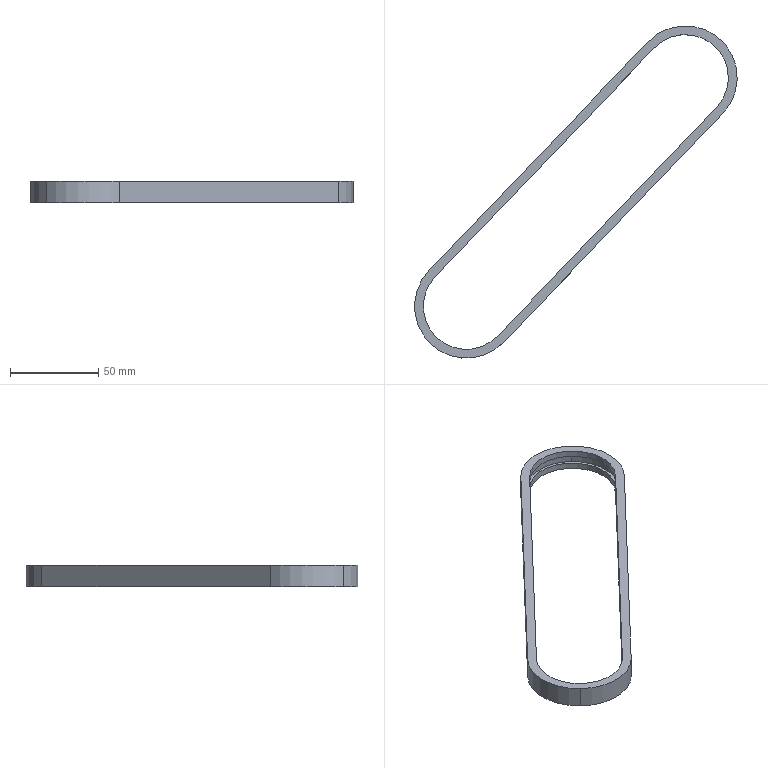Component | SolidWorks | LD101-02-Chain35B-2-1 | 1 solid | 24 faces | box 183.32 x 188.82 x 12 mm | volume 27813 mm3 | cylinder 12 | plane 12 | commonest cylinder face diameters 48.82 x6 52 x3 58.82 x3 | material 45
build123d program:
from build123d import *

# Parameters (mm, degrees)
EXTRUDE_THIN1_DEPTH            = 6
CHAIN_PLATE_GAP_SPROCKET_DEPTH = 2.385


with BuildPart() as part:
    # Sketch1_2 → Extrude-Thin1 (new, symmetric)
    with BuildSketch(Plane.XY):
        with BuildLine():
            Line((90, 29.41), (-90, 29.41))
            ThreePointArc((-90, 29.41), (-119.41, 0), (-90, -29.41))
            Line((-90, -29.41), (90, -29.41))
            ThreePointArc((90, -29.41), (119.41, 0), (90, 29.41))
        make_face()
        with BuildLine():
            Line((90, 24.41), (-90, 24.41))
            ThreePointArc((-90, 24.41), (-114.41, 0), (-90, -24.41))
            Line((-90, -24.41), (90, -24.41))
            ThreePointArc((90, -24.41), (114.41, 0), (90, 24.41))
        make_face(mode=Mode.SUBTRACT)
    extrude(amount=EXTRUDE_THIN1_DEPTH, both=True)

    # Sketch1_2 2 → Chain Plate Gap-Sprocket (cut, symmetric)
    with BuildSketch(Plane.XY):
        with BuildLine():
            Line((90, 26), (-90, 26))
            ThreePointArc((-90, 26), (-116, 0), (-90, -26))
            Line((-90, -26), (90, -26))
            ThreePointArc((90, -26), (116, 0), (90, 26))
        make_face()
        with BuildLine():
            Line((90, 22.82), (-90, 22.82))
            ThreePointArc((-90, 22.82), (-112.82, 0), (-90, -22.82))
            Line((-90, -22.82), (90, -22.82))
            ThreePointArc((90, -22.82), (112.82, 0), (90, 22.82))
        make_face(mode=Mode.SUBTRACT)
    extrude(amount=CHAIN_PLATE_GAP_SPROCKET_DEPTH, both=True, mode=Mode.SUBTRACT)


solid = part.part

# Placed as in the assembly
solid = solid.moved(Location((309.461, -246.897, 314.107), (0, 0, -133.762)))
STEP:
#1=COLOUR_RGB('',0.7922,0.8196,0.9333);
#2=FILL_AREA_STYLE_COLOUR('',#1);
#3=FILL_AREA_STYLE('',(#2));
#4=SURFACE_STYLE_FILL_AREA(#3);
#5=SURFACE_SIDE_STYLE('',(#4));
#6=SURFACE_STYLE_USAGE(.BOTH.,#5);
#7=PRESENTATION_STYLE_ASSIGNMENT((#6));
#8=CARTESIAN_POINT('',(15.342,-6.422,12.273));
#9=VERTEX_POINT('',#8);
#10=CARTESIAN_POINT('',(13.895,-6.453,12.273));
#11=VERTEX_POINT('',#10);
#12=CARTESIAN_POINT('',(14.634,-7.161,12.273));
#13=DIRECTION('',(0.,0.,1.));
#14=DIRECTION('',(-0.6917,-0.7222,0.));
#15=AXIS2_PLACEMENT_3D('',#12,#13,#14);
#16=CIRCLE('',#15,1.024);
#17=EDGE_CURVE('',#9,#11,#16,.T.);
#18=ORIENTED_EDGE('',*,*,#17,.F.);
#19=CARTESIAN_POINT('',(15.342,-6.422,12.46));
#20=VERTEX_POINT('',#19);
#21=CARTESIAN_POINT('',(15.342,-6.422,12.273));
#22=DIRECTION('',(0.,0.,1.));
#23=VECTOR('',#22,39.37);
#24=LINE('',#21,#23);
#25=EDGE_CURVE('',#9,#20,#24,.T.);
#26=ORIENTED_EDGE('',*,*,#25,.T.);
#27=CARTESIAN_POINT('',(13.895,-6.453,12.46));
#28=VERTEX_POINT('',#27);
#29=CARTESIAN_POINT('',(14.634,-7.161,12.46));
#30=DIRECTION('',(0.,0.,1.));
#31=DIRECTION('',(-0.6917,-0.7222,0.));
#32=AXIS2_PLACEMENT_3D('',#29,#30,#31);
#33=CIRCLE('',#32,1.024);
#34=EDGE_CURVE('',#20,#28,#33,.T.);
#35=ORIENTED_EDGE('',*,*,#34,.T.);
#36=CARTESIAN_POINT('',(13.895,-6.453,12.273));
#37=DIRECTION('',(0.,0.,1.));
#38=VECTOR('',#37,39.37);
#39=LINE('',#36,#38);
#40=EDGE_CURVE('',#11,#28,#39,.T.);
#41=ORIENTED_EDGE('',*,*,#40,.F.);
#42=EDGE_LOOP('',(#18,#26,#35,#41));
#43=FACE_OUTER_BOUND('',#42,.T.);
#44=CARTESIAN_POINT('',(14.634,-7.161,12.273));
#45=DIRECTION('',(0.,0.,1.));
#46=DIRECTION('',(0.6917,0.7222,0.));
#47=AXIS2_PLACEMENT_3D('',#44,#45,#46);
#48=CYLINDRICAL_SURFACE('',#47,1.024);
#49=ADVANCED_FACE('',(#43),#48,.F.);
#50=CARTESIAN_POINT('',(9.068,-12.973,12.273));
#51=VERTEX_POINT('',#50);
#52=CARTESIAN_POINT('',(9.039,-11.615,12.273));
#53=VERTEX_POINT('',#52);
#54=CARTESIAN_POINT('',(9.733,-12.279,12.273));
#55=DIRECTION('',(0.,0.,-1.));
#56=DIRECTION('',(-0.6917,-0.7222,0.));
#57=AXIS2_PLACEMENT_3D('',#54,#55,#56);
#58=CIRCLE('',#57,0.961);
#59=EDGE_CURVE('',#51,#53,#58,.T.);
#60=ORIENTED_EDGE('',*,*,#59,.F.);
#61=CARTESIAN_POINT('',(9.068,-12.973,12.13));
#62=VERTEX_POINT('',#61);
#63=CARTESIAN_POINT('',(9.068,-12.973,12.603));
#64=DIRECTION('',(0.,0.,-1.));
#65=VECTOR('',#64,39.37);
#66=LINE('',#63,#65);
#67=EDGE_CURVE('',#51,#62,#66,.T.);
#68=ORIENTED_EDGE('',*,*,#67,.T.);
#69=CARTESIAN_POINT('',(9.039,-11.615,12.13));
#70=VERTEX_POINT('',#69);
#71=CARTESIAN_POINT('',(9.733,-12.279,12.13));
#72=DIRECTION('',(0.,0.,1.));
#73=DIRECTION('',(0.6917,0.7222,0.));
#74=AXIS2_PLACEMENT_3D('',#71,#72,#73);
#75=CIRCLE('',#74,0.961);
#76=EDGE_CURVE('',#70,#62,#75,.T.);
#77=ORIENTED_EDGE('',*,*,#76,.F.);
#78=CARTESIAN_POINT('',(9.039,-11.615,12.603));
#79=DIRECTION('',(0.,0.,-1.));
#80=VECTOR('',#79,39.37);
#81=LINE('',#78,#80);
#82=EDGE_CURVE('',#53,#70,#81,.T.);
#83=ORIENTED_EDGE('',*,*,#82,.F.);
#84=EDGE_LOOP('',(#60,#68,#77,#83));
#85=FACE_OUTER_BOUND('',#84,.T.);
#86=CARTESIAN_POINT('',(9.733,-12.279,12.603));
#87=DIRECTION('',(0.,0.,-1.));
#88=DIRECTION('',(-0.6917,-0.7222,0.));
#89=AXIS2_PLACEMENT_3D('',#86,#87,#88);
#90=CYLINDRICAL_SURFACE('',#89,0.961);
#91=ADVANCED_FACE('',(#85),#90,.F.);
#92=CARTESIAN_POINT('',(8.932,-13.116,12.603));
#93=VERTEX_POINT('',#92);
#94=CARTESIAN_POINT('',(10.569,-13.08,12.603));
#95=VERTEX_POINT('',#94);
#96=CARTESIAN_POINT('',(9.733,-12.279,12.603));
#97=DIRECTION('',(0.,0.,1.));
#98=DIRECTION('',(-0.6917,-0.7222,0.));
#99=AXIS2_PLACEMENT_3D('',#96,#97,#98);
#100=CIRCLE('',#99,1.158);
#101=EDGE_CURVE('',#93,#95,#100,.T.);
#102=ORIENTED_EDGE('',*,*,#101,.F.);
#103=CARTESIAN_POINT('',(8.932,-13.116,12.13));
#104=VERTEX_POINT('',#103);
#105=CARTESIAN_POINT('',(8.932,-13.116,12.603));
#106=DIRECTION('',(0.,0.,-1.));
#107=VECTOR('',#106,39.37);
#108=LINE('',#105,#107);
#109=EDGE_CURVE('',#93,#104,#108,.T.);
#110=ORIENTED_EDGE('',*,*,#109,.T.);
#111=CARTESIAN_POINT('',(10.569,-13.08,12.13));
#112=VERTEX_POINT('',#111);
#113=CARTESIAN_POINT('',(9.733,-12.279,12.13));
#114=DIRECTION('',(0.,0.,1.));
#115=DIRECTION('',(-0.6917,-0.7222,0.));
#116=AXIS2_PLACEMENT_3D('',#113,#114,#115);
#117=CIRCLE('',#116,1.158);
#118=EDGE_CURVE('',#104,#112,#117,.T.);
#119=ORIENTED_EDGE('',*,*,#118,.T.);
#120=CARTESIAN_POINT('',(10.569,-13.08,12.603));
#121=DIRECTION('',(0.,0.,-1.));
#122=VECTOR('',#121,39.37);
#123=LINE('',#120,#122);
#124=EDGE_CURVE('',#95,#112,#123,.T.);
#125=ORIENTED_EDGE('',*,*,#124,.F.);
#126=EDGE_LOOP('',(#102,#110,#119,#125));
#127=FACE_OUTER_BOUND('',#126,.T.);
#128=CARTESIAN_POINT('',(9.733,-12.279,12.603));
#129=DIRECTION('',(0.,0.,-1.));
#130=DIRECTION('',(-0.6917,-0.7222,0.));
#131=AXIS2_PLACEMENT_3D('',#128,#129,#130);
#132=CYLINDRICAL_SURFACE('',#131,1.158);
#133=ADVANCED_FACE('',(#127),#132,.T.);
#134=CARTESIAN_POINT('',(9.039,-11.615,12.603));
#135=VERTEX_POINT('',#134);
#136=CARTESIAN_POINT('',(9.068,-12.973,12.603));
#137=VERTEX_POINT('',#136);
#138=CARTESIAN_POINT('',(9.733,-12.279,12.603));
#139=DIRECTION('',(0.,0.,1.));
#140=DIRECTION('',(0.6917,0.7222,0.));
#141=AXIS2_PLACEMENT_3D('',#138,#139,#140);
#142=CIRCLE('',#141,0.961);
#143=EDGE_CURVE('',#135,#137,#142,.T.);
#144=ORIENTED_EDGE('',*,*,#143,.T.);
#145=CARTESIAN_POINT('',(9.068,-12.973,12.46));
#146=VERTEX_POINT('',#145);
#147=CARTESIAN_POINT('',(9.068,-12.973,12.603));
#148=DIRECTION('',(0.,0.,-1.));
#149=VECTOR('',#148,39.37);
#150=LINE('',#147,#149);
#151=EDGE_CURVE('',#137,#146,#150,.T.);
#152=ORIENTED_EDGE('',*,*,#151,.T.);
#153=CARTESIAN_POINT('',(9.039,-11.615,12.46));
#154=VERTEX_POINT('',#153);
#155=CARTESIAN_POINT('',(9.733,-12.279,12.46));
#156=DIRECTION('',(0.,0.,-1.));
#157=DIRECTION('',(-0.6917,-0.7222,0.));
#158=AXIS2_PLACEMENT_3D('',#155,#156,#157);
#159=CIRCLE('',#158,0.961);
#160=EDGE_CURVE('',#146,#154,#159,.T.);
#161=ORIENTED_EDGE('',*,*,#160,.T.);
#162=CARTESIAN_POINT('',(9.039,-11.615,12.603));
#163=DIRECTION('',(0.,0.,-1.));
#164=VECTOR('',#163,39.37);
#165=LINE('',#162,#164);
#166=EDGE_CURVE('',#135,#154,#165,.T.);
#167=ORIENTED_EDGE('',*,*,#166,.F.);
#168=EDGE_LOOP('',(#144,#152,#161,#167));
#169=FACE_OUTER_BOUND('',#168,.T.);
#170=CARTESIAN_POINT('',(9.733,-12.279,12.603));
#171=DIRECTION('',(0.,0.,-1.));
#172=DIRECTION('',(-0.6917,-0.7222,0.));
#173=AXIS2_PLACEMENT_3D('',#170,#171,#172);
#174=CYLINDRICAL_SURFACE('',#173,0.961);
#175=ADVANCED_FACE('',(#169),#174,.F.);
#176=CARTESIAN_POINT('',(13.94,-6.497,12.603));
#177=VERTEX_POINT('',#176);
#178=CARTESIAN_POINT('',(13.94,-6.497,12.46));
#179=VERTEX_POINT('',#178);
#180=CARTESIAN_POINT('',(13.94,-6.497,12.603));
#181=DIRECTION('',(0.,0.,-1.));
#182=VECTOR('',#181,39.37);
#183=LINE('',#180,#182);
#184=EDGE_CURVE('',#177,#179,#183,.T.);
#185=ORIENTED_EDGE('',*,*,#184,.T.);
#186=CARTESIAN_POINT('',(15.328,-7.826,12.46));
#187=VERTEX_POINT('',#186);
#188=CARTESIAN_POINT('',(14.634,-7.161,12.46));
#189=DIRECTION('',(0.,0.,-1.));
#190=DIRECTION('',(-0.6917,-0.7222,0.));
#191=AXIS2_PLACEMENT_3D('',#188,#189,#190);
#192=CIRCLE('',#191,0.961);
#193=EDGE_CURVE('',#179,#187,#192,.T.);
#194=ORIENTED_EDGE('',*,*,#193,.T.);
#195=CARTESIAN_POINT('',(15.328,-7.826,12.603));
#196=VERTEX_POINT('',#195);
#197=CARTESIAN_POINT('',(15.328,-7.826,12.603));
#198=DIRECTION('',(0.,0.,-1.));
#199=VECTOR('',#198,39.37);
#200=LINE('',#197,#199);
#201=EDGE_CURVE('',#196,#187,#200,.T.);
#202=ORIENTED_EDGE('',*,*,#201,.F.);
#203=CARTESIAN_POINT('',(14.634,-7.161,12.603));
#204=DIRECTION('',(0.,0.,1.));
#205=DIRECTION('',(-0.6917,-0.7222,0.));
#206=AXIS2_PLACEMENT_3D('',#203,#204,#205);
#207=CIRCLE('',#206,0.961);
#208=EDGE_CURVE('',#196,#177,#207,.T.);
#209=ORIENTED_EDGE('',*,*,#208,.T.);
#210=EDGE_LOOP('',(#185,#194,#202,#209));
#211=FACE_OUTER_BOUND('',#210,.T.);
#212=CARTESIAN_POINT('',(14.634,-7.161,12.603));
#213=DIRECTION('',(0.,0.,-1.));
#214=DIRECTION('',(-0.6917,-0.7222,0.));
#215=AXIS2_PLACEMENT_3D('',#212,#213,#214);
#216=CYLINDRICAL_SURFACE('',#215,0.961);
#217=ADVANCED_FACE('',(#211),#216,.F.);
#218=ORIENTED_EDGE('',*,*,#166,.T.);
#219=CARTESIAN_POINT('',(13.94,-6.497,12.46));
#220=DIRECTION('',(0.6917,0.7222,0.));
#221=VECTOR('',#220,39.37);
#222=LINE('',#219,#221);
#223=EDGE_CURVE('',#154,#179,#222,.T.);
#224=ORIENTED_EDGE('',*,*,#223,.T.);
#225=ORIENTED_EDGE('',*,*,#184,.F.);
#226=CARTESIAN_POINT('',(13.94,-6.497,12.603));
#227=DIRECTION('',(-0.6917,-0.7222,0.));
#228=VECTOR('',#227,39.37);
#229=LINE('',#226,#228);
#230=EDGE_CURVE('',#177,#135,#229,.T.);
#231=ORIENTED_EDGE('',*,*,#230,.T.);
#232=EDGE_LOOP('',(#218,#224,#225,#231));
#233=FACE_OUTER_BOUND('',#232,.T.);
#234=CARTESIAN_POINT('',(13.94,-6.497,12.603));
#235=DIRECTION('',(0.7222,-0.6917,0.));
#236=DIRECTION('',(0.,0.,-1.));
#237=AXIS2_PLACEMENT_3D('',#234,#235,#236);
#238=PLANE('',#237);
#239=ADVANCED_FACE('',(#233),#238,.T.);
#240=ORIENTED_EDGE('',*,*,#151,.F.);
#241=CARTESIAN_POINT('',(10.427,-12.944,12.603));
#242=VERTEX_POINT('',#241);
#243=CARTESIAN_POINT('',(9.733,-12.279,12.603));
#244=DIRECTION('',(0.,0.,1.));
#245=DIRECTION('',(0.6917,0.7222,0.));
#246=AXIS2_PLACEMENT_3D('',#243,#244,#245);
#247=CIRCLE('',#246,0.961);
#248=EDGE_CURVE('',#137,#242,#247,.T.);
#249=ORIENTED_EDGE('',*,*,#248,.T.);
#250=CARTESIAN_POINT('',(10.427,-12.944,12.46));
#251=VERTEX_POINT('',#250);
#252=CARTESIAN_POINT('',(10.427,-12.944,12.603));
#253=DIRECTION('',(0.,0.,-1.));
#254=VECTOR('',#253,39.37);
#255=LINE('',#252,#254);
#256=EDGE_CURVE('',#242,#251,#255,.T.);
#257=ORIENTED_EDGE('',*,*,#256,.T.);
#258=CARTESIAN_POINT('',(9.733,-12.279,12.46));
#259=DIRECTION('',(0.,0.,-1.));
#260=DIRECTION('',(-0.6917,-0.7222,0.));
#261=AXIS2_PLACEMENT_3D('',#258,#259,#260);
#262=CIRCLE('',#261,0.961);
#263=EDGE_CURVE('',#251,#146,#262,.T.);
#264=ORIENTED_EDGE('',*,*,#263,.T.);
#265=EDGE_LOOP('',(#240,#249,#257,#264));
#266=FACE_OUTER_BOUND('',#265,.T.);
#267=CARTESIAN_POINT('',(9.733,-12.279,12.603));
#268=DIRECTION('',(0.,0.,-1.));
#269=DIRECTION('',(-0.6917,-0.7222,0.));
#270=AXIS2_PLACEMENT_3D('',#267,#268,#269);
#271=CYLINDRICAL_SURFACE('',#270,0.961);
#272=ADVANCED_FACE('',(#266),#271,.F.);
#273=ORIENTED_EDGE('',*,*,#201,.T.);
#274=CARTESIAN_POINT('',(10.427,-12.944,12.46));
#275=DIRECTION('',(-0.6917,-0.7222,0.));
#276=VECTOR('',#275,39.37);
#277=LINE('',#274,#276);
#278=EDGE_CURVE('',#187,#251,#277,.T.);
#279=ORIENTED_EDGE('',*,*,#278,.T.);
#280=ORIENTED_EDGE('',*,*,#256,.F.);
#281=CARTESIAN_POINT('',(10.427,-12.944,12.603));
#282=DIRECTION('',(0.6917,0.7222,0.));
#283=VECTOR('',#282,39.37);
#284=LINE('',#281,#283);
#285=EDGE_CURVE('',#242,#196,#284,.T.);
#286=ORIENTED_EDGE('',*,*,#285,.T.);
#287=EDGE_LOOP('',(#273,#279,#280,#286));
#288=FACE_OUTER_BOUND('',#287,.T.);
#289=CARTESIAN_POINT('',(10.427,-12.944,12.603));
#290=DIRECTION('',(-0.7222,0.6917,0.));
#291=DIRECTION('',(0.,0.,1.));
#292=AXIS2_PLACEMENT_3D('',#289,#290,#291);
#293=PLANE('',#292);
#294=ADVANCED_FACE('',(#288),#293,.T.);
#295=CARTESIAN_POINT('',(15.471,-7.962,12.603));
#296=VERTEX_POINT('',#295);
#297=CARTESIAN_POINT('',(13.798,-6.36,12.603));
#298=VERTEX_POINT('',#297);
#299=CARTESIAN_POINT('',(14.634,-7.161,12.603));
#300=DIRECTION('',(0.,0.,1.));
#301=DIRECTION('',(-0.6917,-0.7222,0.));
#302=AXIS2_PLACEMENT_3D('',#299,#300,#301);
#303=CIRCLE('',#302,1.158);
#304=EDGE_CURVE('',#296,#298,#303,.T.);
#305=ORIENTED_EDGE('',*,*,#304,.T.);
#306=CARTESIAN_POINT('',(8.896,-11.479,12.603));
#307=VERTEX_POINT('',#306);
#308=CARTESIAN_POINT('',(13.798,-6.36,12.603));
#309=DIRECTION('',(-0.6917,-0.7222,0.));
#310=VECTOR('',#309,39.37);
#311=LINE('',#308,#310);
#312=EDGE_CURVE('',#298,#307,#311,.T.);
#313=ORIENTED_EDGE('',*,*,#312,.T.);
#314=CARTESIAN_POINT('',(9.733,-12.279,12.603));
#315=DIRECTION('',(0.,0.,1.));
#316=DIRECTION('',(-0.6917,-0.7222,0.));
#317=AXIS2_PLACEMENT_3D('',#314,#315,#316);
#318=CIRCLE('',#317,1.158);
#319=EDGE_CURVE('',#307,#93,#318,.T.);
#320=ORIENTED_EDGE('',*,*,#319,.T.);
#321=ORIENTED_EDGE('',*,*,#101,.T.);
#322=CARTESIAN_POINT('',(15.471,-7.962,12.603));
#323=DIRECTION('',(0.6917,0.7222,0.));
#324=VECTOR('',#323,39.37);
#325=LINE('',#322,#324);
#326=EDGE_CURVE('',#95,#296,#325,.T.);
#327=ORIENTED_EDGE('',*,*,#326,.T.);
#328=EDGE_LOOP('',(#305,#313,#320,#321,#327));
#329=FACE_OUTER_BOUND('',#328,.T.);
#330=ORIENTED_EDGE('',*,*,#208,.F.);
#331=ORIENTED_EDGE('',*,*,#285,.F.);
#332=ORIENTED_EDGE('',*,*,#248,.F.);
#333=ORIENTED_EDGE('',*,*,#143,.F.);
#334=ORIENTED_EDGE('',*,*,#230,.F.);
#335=EDGE_LOOP('',(#330,#331,#332,#333,#334));
#336=FACE_BOUND('',#335,.T.);
#337=CARTESIAN_POINT('',(14.634,-7.161,12.603));
#338=DIRECTION('',(0.,0.,-1.));
#339=DIRECTION('',(-0.6917,-0.7222,0.));
#340=AXIS2_PLACEMENT_3D('',#337,#338,#339);
#341=PLANE('',#340);
#342=ADVANCED_FACE('',(#329,#336),#341,.F.);
#343=CARTESIAN_POINT('',(15.471,-7.962,12.13));
#344=VERTEX_POINT('',#343);
#345=CARTESIAN_POINT('',(13.798,-6.36,12.13));
#346=VERTEX_POINT('',#345);
#347=CARTESIAN_POINT('',(14.634,-7.161,12.13));
#348=DIRECTION('',(0.,0.,1.));
#349=DIRECTION('',(-0.6917,-0.7222,0.));
#350=AXIS2_PLACEMENT_3D('',#347,#348,#349);
#351=CIRCLE('',#350,1.158);
#352=EDGE_CURVE('',#344,#346,#351,.T.);
#353=ORIENTED_EDGE('',*,*,#352,.F.);
#354=CARTESIAN_POINT('',(15.471,-7.962,12.13));
#355=DIRECTION('',(0.6917,0.7222,0.));
#356=VECTOR('',#355,39.37);
#357=LINE('',#354,#356);
#358=EDGE_CURVE('',#112,#344,#357,.T.);
#359=ORIENTED_EDGE('',*,*,#358,.F.);
#360=ORIENTED_EDGE('',*,*,#118,.F.);
#361=CARTESIAN_POINT('',(8.896,-11.479,12.13));
#362=VERTEX_POINT('',#361);
#363=CARTESIAN_POINT('',(9.733,-12.279,12.13));
#364=DIRECTION('',(0.,0.,1.));
#365=DIRECTION('',(-0.6917,-0.7222,0.));
#366=AXIS2_PLACEMENT_3D('',#363,#364,#365);
#367=CIRCLE('',#366,1.158);
#368=EDGE_CURVE('',#362,#104,#367,.T.);
#369=ORIENTED_EDGE('',*,*,#368,.F.);
#370=CARTESIAN_POINT('',(13.798,-6.36,12.13));
#371=DIRECTION('',(-0.6917,-0.7222,0.));
#372=VECTOR('',#371,39.37);
#373=LINE('',#370,#372);
#374=EDGE_CURVE('',#346,#362,#373,.T.);
#375=ORIENTED_EDGE('',*,*,#374,.F.);
#376=EDGE_LOOP('',(#353,#359,#360,#369,#375));
#377=FACE_OUTER_BOUND('',#376,.T.);
#378=CARTESIAN_POINT('',(10.427,-12.944,12.13));
#379=VERTEX_POINT('',#378);
#380=CARTESIAN_POINT('',(15.328,-7.826,12.13));
#381=VERTEX_POINT('',#380);
#382=CARTESIAN_POINT('',(10.427,-12.944,12.13));
#383=DIRECTION('',(0.6917,0.7222,0.));
#384=VECTOR('',#383,39.37);
#385=LINE('',#382,#384);
#386=EDGE_CURVE('',#379,#381,#385,.T.);
#387=ORIENTED_EDGE('',*,*,#386,.T.);
#388=CARTESIAN_POINT('',(13.94,-6.497,12.13));
#389=VERTEX_POINT('',#388);
#390=CARTESIAN_POINT('',(14.634,-7.161,12.13));
#391=DIRECTION('',(0.,0.,1.));
#392=DIRECTION('',(-0.6917,-0.7222,0.));
#393=AXIS2_PLACEMENT_3D('',#390,#391,#392);
#394=CIRCLE('',#393,0.961);
#395=EDGE_CURVE('',#381,#389,#394,.T.);
#396=ORIENTED_EDGE('',*,*,#395,.T.);
#397=CARTESIAN_POINT('',(13.94,-6.497,12.13));
#398=DIRECTION('',(-0.6917,-0.7222,0.));
#399=VECTOR('',#398,39.37);
#400=LINE('',#397,#399);
#401=EDGE_CURVE('',#389,#70,#400,.T.);
#402=ORIENTED_EDGE('',*,*,#401,.T.);
#403=ORIENTED_EDGE('',*,*,#76,.T.);
#404=CARTESIAN_POINT('',(9.733,-12.279,12.13));
#405=DIRECTION('',(0.,0.,1.));
#406=DIRECTION('',(0.6917,0.7222,0.));
#407=AXIS2_PLACEMENT_3D('',#404,#405,#406);
#408=CIRCLE('',#407,0.961);
#409=EDGE_CURVE('',#62,#379,#408,.T.);
#410=ORIENTED_EDGE('',*,*,#409,.T.);
#411=EDGE_LOOP('',(#387,#396,#402,#403,#410));
#412=FACE_BOUND('',#411,.T.);
#413=CARTESIAN_POINT('',(14.634,-7.161,12.13));
#414=DIRECTION('',(0.,0.,-1.));
#415=DIRECTION('',(-0.6917,-0.7222,0.));
#416=AXIS2_PLACEMENT_3D('',#413,#414,#415);
#417=PLANE('',#416);
#418=ADVANCED_FACE('',(#377,#412),#417,.T.);
#419=ORIENTED_EDGE('',*,*,#352,.T.);
#420=CARTESIAN_POINT('',(13.798,-6.36,12.603));
#421=DIRECTION('',(0.,0.,-1.));
#422=VECTOR('',#421,39.37);
#423=LINE('',#420,#422);
#424=EDGE_CURVE('',#298,#346,#423,.T.);
#425=ORIENTED_EDGE('',*,*,#424,.F.);
#426=ORIENTED_EDGE('',*,*,#304,.F.);
#427=CARTESIAN_POINT('',(15.471,-7.962,12.603));
#428=DIRECTION('',(0.,0.,-1.));
#429=VECTOR('',#428,39.37);
#430=LINE('',#427,#429);
#431=EDGE_CURVE('',#296,#344,#430,.T.);
#432=ORIENTED_EDGE('',*,*,#431,.T.);
#433=EDGE_LOOP('',(#419,#425,#426,#432));
#434=FACE_OUTER_BOUND('',#433,.T.);
#435=CARTESIAN_POINT('',(14.634,-7.161,12.603));
#436=DIRECTION('',(0.,0.,-1.));
#437=DIRECTION('',(-0.6917,-0.7222,0.));
#438=AXIS2_PLACEMENT_3D('',#435,#436,#437);
#439=CYLINDRICAL_SURFACE('',#438,1.158);
#440=ADVANCED_FACE('',(#434),#439,.T.);
#441=ORIENTED_EDGE('',*,*,#374,.T.);
#442=CARTESIAN_POINT('',(8.896,-11.479,12.603));
#443=DIRECTION('',(0.,0.,-1.));
#444=VECTOR('',#443,39.37);
#445=LINE('',#442,#444);
#446=EDGE_CURVE('',#307,#362,#445,.T.);
#447=ORIENTED_EDGE('',*,*,#446,.F.);
#448=ORIENTED_EDGE('',*,*,#312,.F.);
#449=ORIENTED_EDGE('',*,*,#424,.T.);
#450=EDGE_LOOP('',(#441,#447,#448,#449));
#451=FACE_OUTER_BOUND('',#450,.T.);
#452=CARTESIAN_POINT('',(13.798,-6.36,12.603));
#453=DIRECTION('',(0.7222,-0.6917,0.));
#454=DIRECTION('',(0.,0.,-1.));
#455=AXIS2_PLACEMENT_3D('',#452,#453,#454);
#456=PLANE('',#455);
#457=ADVANCED_FACE('',(#451),#456,.F.);
#458=ORIENTED_EDGE('',*,*,#109,.F.);
#459=ORIENTED_EDGE('',*,*,#319,.F.);
#460=ORIENTED_EDGE('',*,*,#446,.T.);
#461=ORIENTED_EDGE('',*,*,#368,.T.);
#462=EDGE_LOOP('',(#458,#459,#460,#461));
#463=FACE_OUTER_BOUND('',#462,.T.);
#464=CARTESIAN_POINT('',(9.733,-12.279,12.603));
#465=DIRECTION('',(0.,0.,-1.));
#466=DIRECTION('',(-0.6917,-0.7222,0.));
#467=AXIS2_PLACEMENT_3D('',#464,#465,#466);
#468=CYLINDRICAL_SURFACE('',#467,1.158);
#469=ADVANCED_FACE('',(#463),#468,.T.);
#470=ORIENTED_EDGE('',*,*,#358,.T.);
#471=ORIENTED_EDGE('',*,*,#431,.F.);
#472=ORIENTED_EDGE('',*,*,#326,.F.);
#473=ORIENTED_EDGE('',*,*,#124,.T.);
#474=EDGE_LOOP('',(#470,#471,#472,#473));
#475=FACE_OUTER_BOUND('',#474,.T.);
#476=CARTESIAN_POINT('',(15.471,-7.962,12.603));
#477=DIRECTION('',(-0.7222,0.6917,0.));
#478=DIRECTION('',(0.,0.,1.));
#479=AXIS2_PLACEMENT_3D('',#476,#477,#478);
#480=PLANE('',#479);
#481=ADVANCED_FACE('',(#475),#480,.F.);
#482=CARTESIAN_POINT('',(13.94,-6.497,12.273));
#483=VERTEX_POINT('',#482);
#484=CARTESIAN_POINT('',(15.328,-7.826,12.273));
#485=VERTEX_POINT('',#484);
#486=CARTESIAN_POINT('',(14.634,-7.161,12.273));
#487=DIRECTION('',(0.,0.,-1.));
#488=DIRECTION('',(-0.6917,-0.7222,0.));
#489=AXIS2_PLACEMENT_3D('',#486,#487,#488);
#490=CIRCLE('',#489,0.961);
#491=EDGE_CURVE('',#483,#485,#490,.T.);
#492=ORIENTED_EDGE('',*,*,#491,.F.);
#493=CARTESIAN_POINT('',(13.94,-6.497,12.603));
#494=DIRECTION('',(0.,0.,-1.));
#495=VECTOR('',#494,39.37);
#496=LINE('',#493,#495);
#497=EDGE_CURVE('',#483,#389,#496,.T.);
#498=ORIENTED_EDGE('',*,*,#497,.T.);
#499=ORIENTED_EDGE('',*,*,#395,.F.);
#500=CARTESIAN_POINT('',(15.328,-7.826,12.603));
#501=DIRECTION('',(0.,0.,-1.));
#502=VECTOR('',#501,39.37);
#503=LINE('',#500,#502);
#504=EDGE_CURVE('',#485,#381,#503,.T.);
#505=ORIENTED_EDGE('',*,*,#504,.F.);
#506=EDGE_LOOP('',(#492,#498,#499,#505));
#507=FACE_OUTER_BOUND('',#506,.T.);
#508=CARTESIAN_POINT('',(14.634,-7.161,12.603));
#509=DIRECTION('',(0.,0.,-1.));
#510=DIRECTION('',(-0.6917,-0.7222,0.));
#511=AXIS2_PLACEMENT_3D('',#508,#509,#510);
#512=CYLINDRICAL_SURFACE('',#511,0.961);
#513=ADVANCED_FACE('',(#507),#512,.F.);
#514=CARTESIAN_POINT('',(13.94,-6.497,12.273));
#515=DIRECTION('',(0.6917,0.7222,0.));
#516=VECTOR('',#515,39.37);
#517=LINE('',#514,#516);
#518=EDGE_CURVE('',#53,#483,#517,.T.);
#519=ORIENTED_EDGE('',*,*,#518,.F.);
#520=ORIENTED_EDGE('',*,*,#82,.T.);
#521=ORIENTED_EDGE('',*,*,#401,.F.);
#522=ORIENTED_EDGE('',*,*,#497,.F.);
#523=EDGE_LOOP('',(#519,#520,#521,#522));
#524=FACE_OUTER_BOUND('',#523,.T.);
#525=CARTESIAN_POINT('',(13.94,-6.497,12.603));
#526=DIRECTION('',(0.7222,-0.6917,0.));
#527=DIRECTION('',(0.,0.,-1.));
#528=AXIS2_PLACEMENT_3D('',#525,#526,#527);
#529=PLANE('',#528);
#530=ADVANCED_FACE('',(#524),#529,.T.);
#531=ORIENTED_EDGE('',*,*,#67,.F.);
#532=CARTESIAN_POINT('',(10.427,-12.944,12.273));
#533=VERTEX_POINT('',#532);
#534=CARTESIAN_POINT('',(9.733,-12.279,12.273));
#535=DIRECTION('',(0.,0.,-1.));
#536=DIRECTION('',(-0.6917,-0.7222,0.));
#537=AXIS2_PLACEMENT_3D('',#534,#535,#536);
#538=CIRCLE('',#537,0.961);
#539=EDGE_CURVE('',#533,#51,#538,.T.);
#540=ORIENTED_EDGE('',*,*,#539,.F.);
#541=CARTESIAN_POINT('',(10.427,-12.944,12.603));
#542=DIRECTION('',(0.,0.,-1.));
#543=VECTOR('',#542,39.37);
#544=LINE('',#541,#543);
#545=EDGE_CURVE('',#533,#379,#544,.T.);
#546=ORIENTED_EDGE('',*,*,#545,.T.);
#547=ORIENTED_EDGE('',*,*,#409,.F.);
#548=EDGE_LOOP('',(#531,#540,#546,#547));
#549=FACE_OUTER_BOUND('',#548,.T.);
#550=CARTESIAN_POINT('',(9.733,-12.279,12.603));
#551=DIRECTION('',(0.,0.,-1.));
#552=DIRECTION('',(-0.6917,-0.7222,0.));
#553=AXIS2_PLACEMENT_3D('',#550,#551,#552);
#554=CYLINDRICAL_SURFACE('',#553,0.961);
#555=ADVANCED_FACE('',(#549),#554,.F.);
#556=CARTESIAN_POINT('',(10.427,-12.944,12.273));
#557=DIRECTION('',(-0.6917,-0.7222,0.));
#558=VECTOR('',#557,39.37);
#559=LINE('',#556,#558);
#560=EDGE_CURVE('',#485,#533,#559,.T.);
#561=ORIENTED_EDGE('',*,*,#560,.F.);
#562=ORIENTED_EDGE('',*,*,#504,.T.);
#563=ORIENTED_EDGE('',*,*,#386,.F.);
#564=ORIENTED_EDGE('',*,*,#545,.F.);
#565=EDGE_LOOP('',(#561,#562,#563,#564));
#566=FACE_OUTER_BOUND('',#565,.T.);
#567=CARTESIAN_POINT('',(10.427,-12.944,12.603));
#568=DIRECTION('',(-0.7222,0.6917,0.));
#569=DIRECTION('',(0.,0.,1.));
#570=AXIS2_PLACEMENT_3D('',#567,#568,#569);
#571=PLANE('',#570);
#572=ADVANCED_FACE('',(#566),#571,.T.);
#573=ORIENTED_EDGE('',*,*,#25,.F.);
#574=CARTESIAN_POINT('',(15.374,-7.869,12.273));
#575=VERTEX_POINT('',#574);
#576=CARTESIAN_POINT('',(14.634,-7.161,12.273));
#577=DIRECTION('',(0.,0.,1.));
#578=DIRECTION('',(-0.6917,-0.7222,0.));
#579=AXIS2_PLACEMENT_3D('',#576,#577,#578);
#580=CIRCLE('',#579,1.024);
#581=EDGE_CURVE('',#575,#9,#580,.T.);
#582=ORIENTED_EDGE('',*,*,#581,.F.);
#583=CARTESIAN_POINT('',(15.374,-7.869,12.46));
#584=VERTEX_POINT('',#583);
#585=CARTESIAN_POINT('',(15.374,-7.869,12.273));
#586=DIRECTION('',(0.,0.,1.));
#587=VECTOR('',#586,39.37);
#588=LINE('',#585,#587);
#589=EDGE_CURVE('',#575,#584,#588,.T.);
#590=ORIENTED_EDGE('',*,*,#589,.T.);
#591=CARTESIAN_POINT('',(14.634,-7.161,12.46));
#592=DIRECTION('',(0.,0.,1.));
#593=DIRECTION('',(-0.6917,-0.7222,0.));
#594=AXIS2_PLACEMENT_3D('',#591,#592,#593);
#595=CIRCLE('',#594,1.024);
#596=EDGE_CURVE('',#584,#20,#595,.T.);
#597=ORIENTED_EDGE('',*,*,#596,.T.);
#598=EDGE_LOOP('',(#573,#582,#590,#597));
#599=FACE_OUTER_BOUND('',#598,.T.);
#600=CARTESIAN_POINT('',(14.634,-7.161,12.273));
#601=DIRECTION('',(0.,0.,1.));
#602=DIRECTION('',(0.6917,0.7222,0.));
#603=AXIS2_PLACEMENT_3D('',#600,#601,#602);
#604=CYLINDRICAL_SURFACE('',#603,1.024);
#605=ADVANCED_FACE('',(#599),#604,.F.);
#606=CARTESIAN_POINT('',(10.472,-12.987,12.46));
#607=VERTEX_POINT('',#606);
#608=CARTESIAN_POINT('',(15.374,-7.869,12.46));
#609=DIRECTION('',(0.6917,0.7222,0.));
#610=VECTOR('',#609,39.37);
#611=LINE('',#608,#610);
#612=EDGE_CURVE('',#607,#584,#611,.T.);
#613=ORIENTED_EDGE('',*,*,#612,.T.);
#614=ORIENTED_EDGE('',*,*,#589,.F.);
#615=CARTESIAN_POINT('',(10.472,-12.987,12.273));
#616=VERTEX_POINT('',#615);
#617=CARTESIAN_POINT('',(15.374,-7.869,12.273));
#618=DIRECTION('',(0.6917,0.7222,0.));
#619=VECTOR('',#618,39.37);
#620=LINE('',#617,#619);
#621=EDGE_CURVE('',#616,#575,#620,.T.);
#622=ORIENTED_EDGE('',*,*,#621,.F.);
#623=CARTESIAN_POINT('',(10.472,-12.987,12.273));
#624=DIRECTION('',(0.,0.,1.));
#625=VECTOR('',#624,39.37);
#626=LINE('',#623,#625);
#627=EDGE_CURVE('',#616,#607,#626,.T.);
#628=ORIENTED_EDGE('',*,*,#627,.T.);
#629=EDGE_LOOP('',(#613,#614,#622,#628));
#630=FACE_OUTER_BOUND('',#629,.T.);
#631=CARTESIAN_POINT('',(15.374,-7.869,12.273));
#632=DIRECTION('',(0.7222,-0.6917,0.));
#633=DIRECTION('',(0.,0.,-1.));
#634=AXIS2_PLACEMENT_3D('',#631,#632,#633);
#635=PLANE('',#634);
#636=ADVANCED_FACE('',(#630),#635,.F.);
#637=CARTESIAN_POINT('',(8.993,-11.571,12.46));
#638=VERTEX_POINT('',#637);
#639=CARTESIAN_POINT('',(9.733,-12.279,12.46));
#640=DIRECTION('',(0.,0.,1.));
#641=DIRECTION('',(-0.6917,-0.7222,0.));
#642=AXIS2_PLACEMENT_3D('',#639,#640,#641);
#643=CIRCLE('',#642,1.024);
#644=EDGE_CURVE('',#638,#607,#643,.T.);
#645=ORIENTED_EDGE('',*,*,#644,.T.);
#646=ORIENTED_EDGE('',*,*,#627,.F.);
#647=CARTESIAN_POINT('',(8.993,-11.571,12.273));
#648=VERTEX_POINT('',#647);
#649=CARTESIAN_POINT('',(9.733,-12.279,12.273));
#650=DIRECTION('',(0.,0.,1.));
#651=DIRECTION('',(-0.6917,-0.7222,0.));
#652=AXIS2_PLACEMENT_3D('',#649,#650,#651);
#653=CIRCLE('',#652,1.024);
#654=EDGE_CURVE('',#648,#616,#653,.T.);
#655=ORIENTED_EDGE('',*,*,#654,.F.);
#656=CARTESIAN_POINT('',(8.993,-11.571,12.273));
#657=DIRECTION('',(0.,0.,1.));
#658=VECTOR('',#657,39.37);
#659=LINE('',#656,#658);
#660=EDGE_CURVE('',#648,#638,#659,.T.);
#661=ORIENTED_EDGE('',*,*,#660,.T.);
#662=EDGE_LOOP('',(#645,#646,#655,#661));
#663=FACE_OUTER_BOUND('',#662,.T.);
#664=CARTESIAN_POINT('',(9.733,-12.279,12.273));
#665=DIRECTION('',(0.,0.,1.));
#666=DIRECTION('',(0.6917,0.7222,0.));
#667=AXIS2_PLACEMENT_3D('',#664,#665,#666);
#668=CYLINDRICAL_SURFACE('',#667,1.024);
#669=ADVANCED_FACE('',(#663),#668,.F.);
#670=CARTESIAN_POINT('',(13.895,-6.453,12.46));
#671=DIRECTION('',(-0.6917,-0.7222,0.));
#672=VECTOR('',#671,39.37);
#673=LINE('',#670,#672);
#674=EDGE_CURVE('',#28,#638,#673,.T.);
#675=ORIENTED_EDGE('',*,*,#674,.T.);
#676=ORIENTED_EDGE('',*,*,#660,.F.);
#677=CARTESIAN_POINT('',(13.895,-6.453,12.273));
#678=DIRECTION('',(-0.6917,-0.7222,0.));
#679=VECTOR('',#678,39.37);
#680=LINE('',#677,#679);
#681=EDGE_CURVE('',#11,#648,#680,.T.);
#682=ORIENTED_EDGE('',*,*,#681,.F.);
#683=ORIENTED_EDGE('',*,*,#40,.T.);
#684=EDGE_LOOP('',(#675,#676,#682,#683));
#685=FACE_OUTER_BOUND('',#684,.T.);
#686=CARTESIAN_POINT('',(13.895,-6.453,12.273));
#687=DIRECTION('',(-0.7222,0.6917,0.));
#688=DIRECTION('',(0.,0.,1.));
#689=AXIS2_PLACEMENT_3D('',#686,#687,#688);
#690=PLANE('',#689);
#691=ADVANCED_FACE('',(#685),#690,.F.);
#692=ORIENTED_EDGE('',*,*,#491,.T.);
#693=ORIENTED_EDGE('',*,*,#560,.T.);
#694=ORIENTED_EDGE('',*,*,#539,.T.);
#695=ORIENTED_EDGE('',*,*,#59,.T.);
#696=ORIENTED_EDGE('',*,*,#518,.T.);
#697=EDGE_LOOP('',(#692,#693,#694,#695,#696));
#698=FACE_BOUND('',#697,.T.);
#699=ORIENTED_EDGE('',*,*,#581,.T.);
#700=ORIENTED_EDGE('',*,*,#17,.T.);
#701=ORIENTED_EDGE('',*,*,#681,.T.);
#702=ORIENTED_EDGE('',*,*,#654,.T.);
#703=ORIENTED_EDGE('',*,*,#621,.T.);
#704=EDGE_LOOP('',(#699,#700,#701,#702,#703));
#705=FACE_OUTER_BOUND('',#704,.T.);
#706=CARTESIAN_POINT('',(14.634,-7.161,12.273));
#707=DIRECTION('',(0.,0.,-1.));
#708=DIRECTION('',(-0.6917,-0.7222,0.));
#709=AXIS2_PLACEMENT_3D('',#706,#707,#708);
#710=PLANE('',#709);
#711=ADVANCED_FACE('',(#698,#705),#710,.F.);
#712=ORIENTED_EDGE('',*,*,#223,.F.);
#713=ORIENTED_EDGE('',*,*,#160,.F.);
#714=ORIENTED_EDGE('',*,*,#263,.F.);
#715=ORIENTED_EDGE('',*,*,#278,.F.);
#716=ORIENTED_EDGE('',*,*,#193,.F.);
#717=EDGE_LOOP('',(#712,#713,#714,#715,#716));
#718=FACE_BOUND('',#717,.T.);
#719=ORIENTED_EDGE('',*,*,#596,.F.);
#720=ORIENTED_EDGE('',*,*,#612,.F.);
#721=ORIENTED_EDGE('',*,*,#644,.F.);
#722=ORIENTED_EDGE('',*,*,#674,.F.);
#723=ORIENTED_EDGE('',*,*,#34,.F.);
#724=EDGE_LOOP('',(#719,#720,#721,#722,#723));
#725=FACE_OUTER_BOUND('',#724,.T.);
#726=CARTESIAN_POINT('',(14.634,-7.161,12.46));
#727=DIRECTION('',(0.,0.,-1.));
#728=DIRECTION('',(-0.6917,-0.7222,0.));
#729=AXIS2_PLACEMENT_3D('',#726,#727,#728);
#730=PLANE('',#729);
#731=ADVANCED_FACE('',(#718,#725),#730,.T.);
#732=CLOSED_SHELL('',(#49,#91,#133,#175,#217,#239,#272,#294,#342,#418,#440,#457,#469,#481,#513,#530,#555,#572,#605,#636,#669,#691,#711,#731));
#733=MANIFOLD_SOLID_BREP('',#732);
#734=STYLED_ITEM('',(#7),#733);
#735=(LENGTH_UNIT()NAMED_UNIT(*)SI_UNIT($,.METRE.));
#736=LENGTH_MEASURE_WITH_UNIT(LENGTH_MEASURE(0.0254),#735);
#737=DIMENSIONAL_EXPONENTS(1.,0.,0.,0.,0.,0.,0.);
#738=(CONVERSION_BASED_UNIT('',#736)LENGTH_UNIT()NAMED_UNIT(#737));
#739=UNCERTAINTY_MEASURE_WITH_UNIT(LENGTH_MEASURE(0.00001),#738,'','');
#740=(NAMED_UNIT(*)PLANE_ANGLE_UNIT()SI_UNIT($,.RADIAN.));
#741=(NAMED_UNIT(*)SI_UNIT($,.STERADIAN.)SOLID_ANGLE_UNIT());
#742=(GEOMETRIC_REPRESENTATION_CONTEXT(3)GLOBAL_UNCERTAINTY_ASSIGNED_CONTEXT((#739))GLOBAL_UNIT_ASSIGNED_CONTEXT((#738,#740,#741))REPRESENTATION_CONTEXT('',''));
#743=MECHANICAL_DESIGN_GEOMETRIC_PRESENTATION_REPRESENTATION('',(#734),#742);
#744=CARTESIAN_POINT('',(0.,0.,0.));
#745=DIRECTION('',(0.,0.,1.));
#746=DIRECTION('',(1.,0.,0.));
#747=AXIS2_PLACEMENT_3D('',#744,#745,#746);
#748=(LENGTH_UNIT()NAMED_UNIT(*)SI_UNIT($,.METRE.));
#749=LENGTH_MEASURE_WITH_UNIT(LENGTH_MEASURE(0.0254),#748);
#750=DIMENSIONAL_EXPONENTS(1.,0.,0.,0.,0.,0.,0.);
#751=(CONVERSION_BASED_UNIT('',#749)LENGTH_UNIT()NAMED_UNIT(#750));
#752=UNCERTAINTY_MEASURE_WITH_UNIT(LENGTH_MEASURE(0.00001),#751,'','');
#753=(NAMED_UNIT(*)PLANE_ANGLE_UNIT()SI_UNIT($,.RADIAN.));
#754=(NAMED_UNIT(*)SI_UNIT($,.STERADIAN.)SOLID_ANGLE_UNIT());
#755=(GEOMETRIC_REPRESENTATION_CONTEXT(3)GLOBAL_UNCERTAINTY_ASSIGNED_CONTEXT((#752))GLOBAL_UNIT_ASSIGNED_CONTEXT((#751,#753,#754))REPRESENTATION_CONTEXT('',''));
#756=ADVANCED_BREP_SHAPE_REPRESENTATION('',(#733,#747),#755);
#757=PRESENTATION_LAYER_ASSIGNMENT('','',(#734));